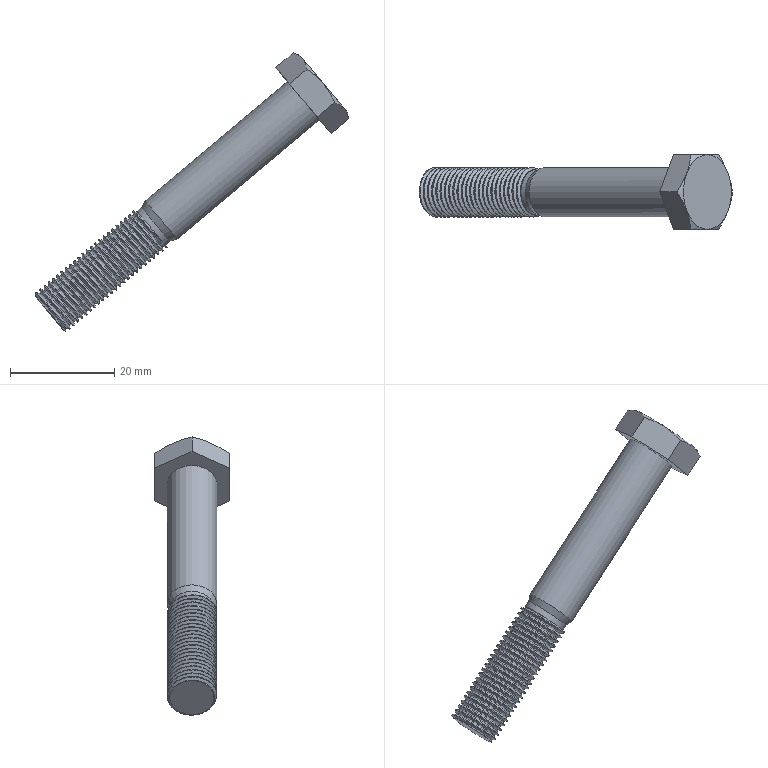Component | NX | KINGPINBOLT | 1 solid | 24 faces | volume 5166 mm3 | plane 10 | cone 8 | cylinder 4 | spline 2 | commonest cylinder face diameters 9.525 x2 8.46 x1 8.467 x1